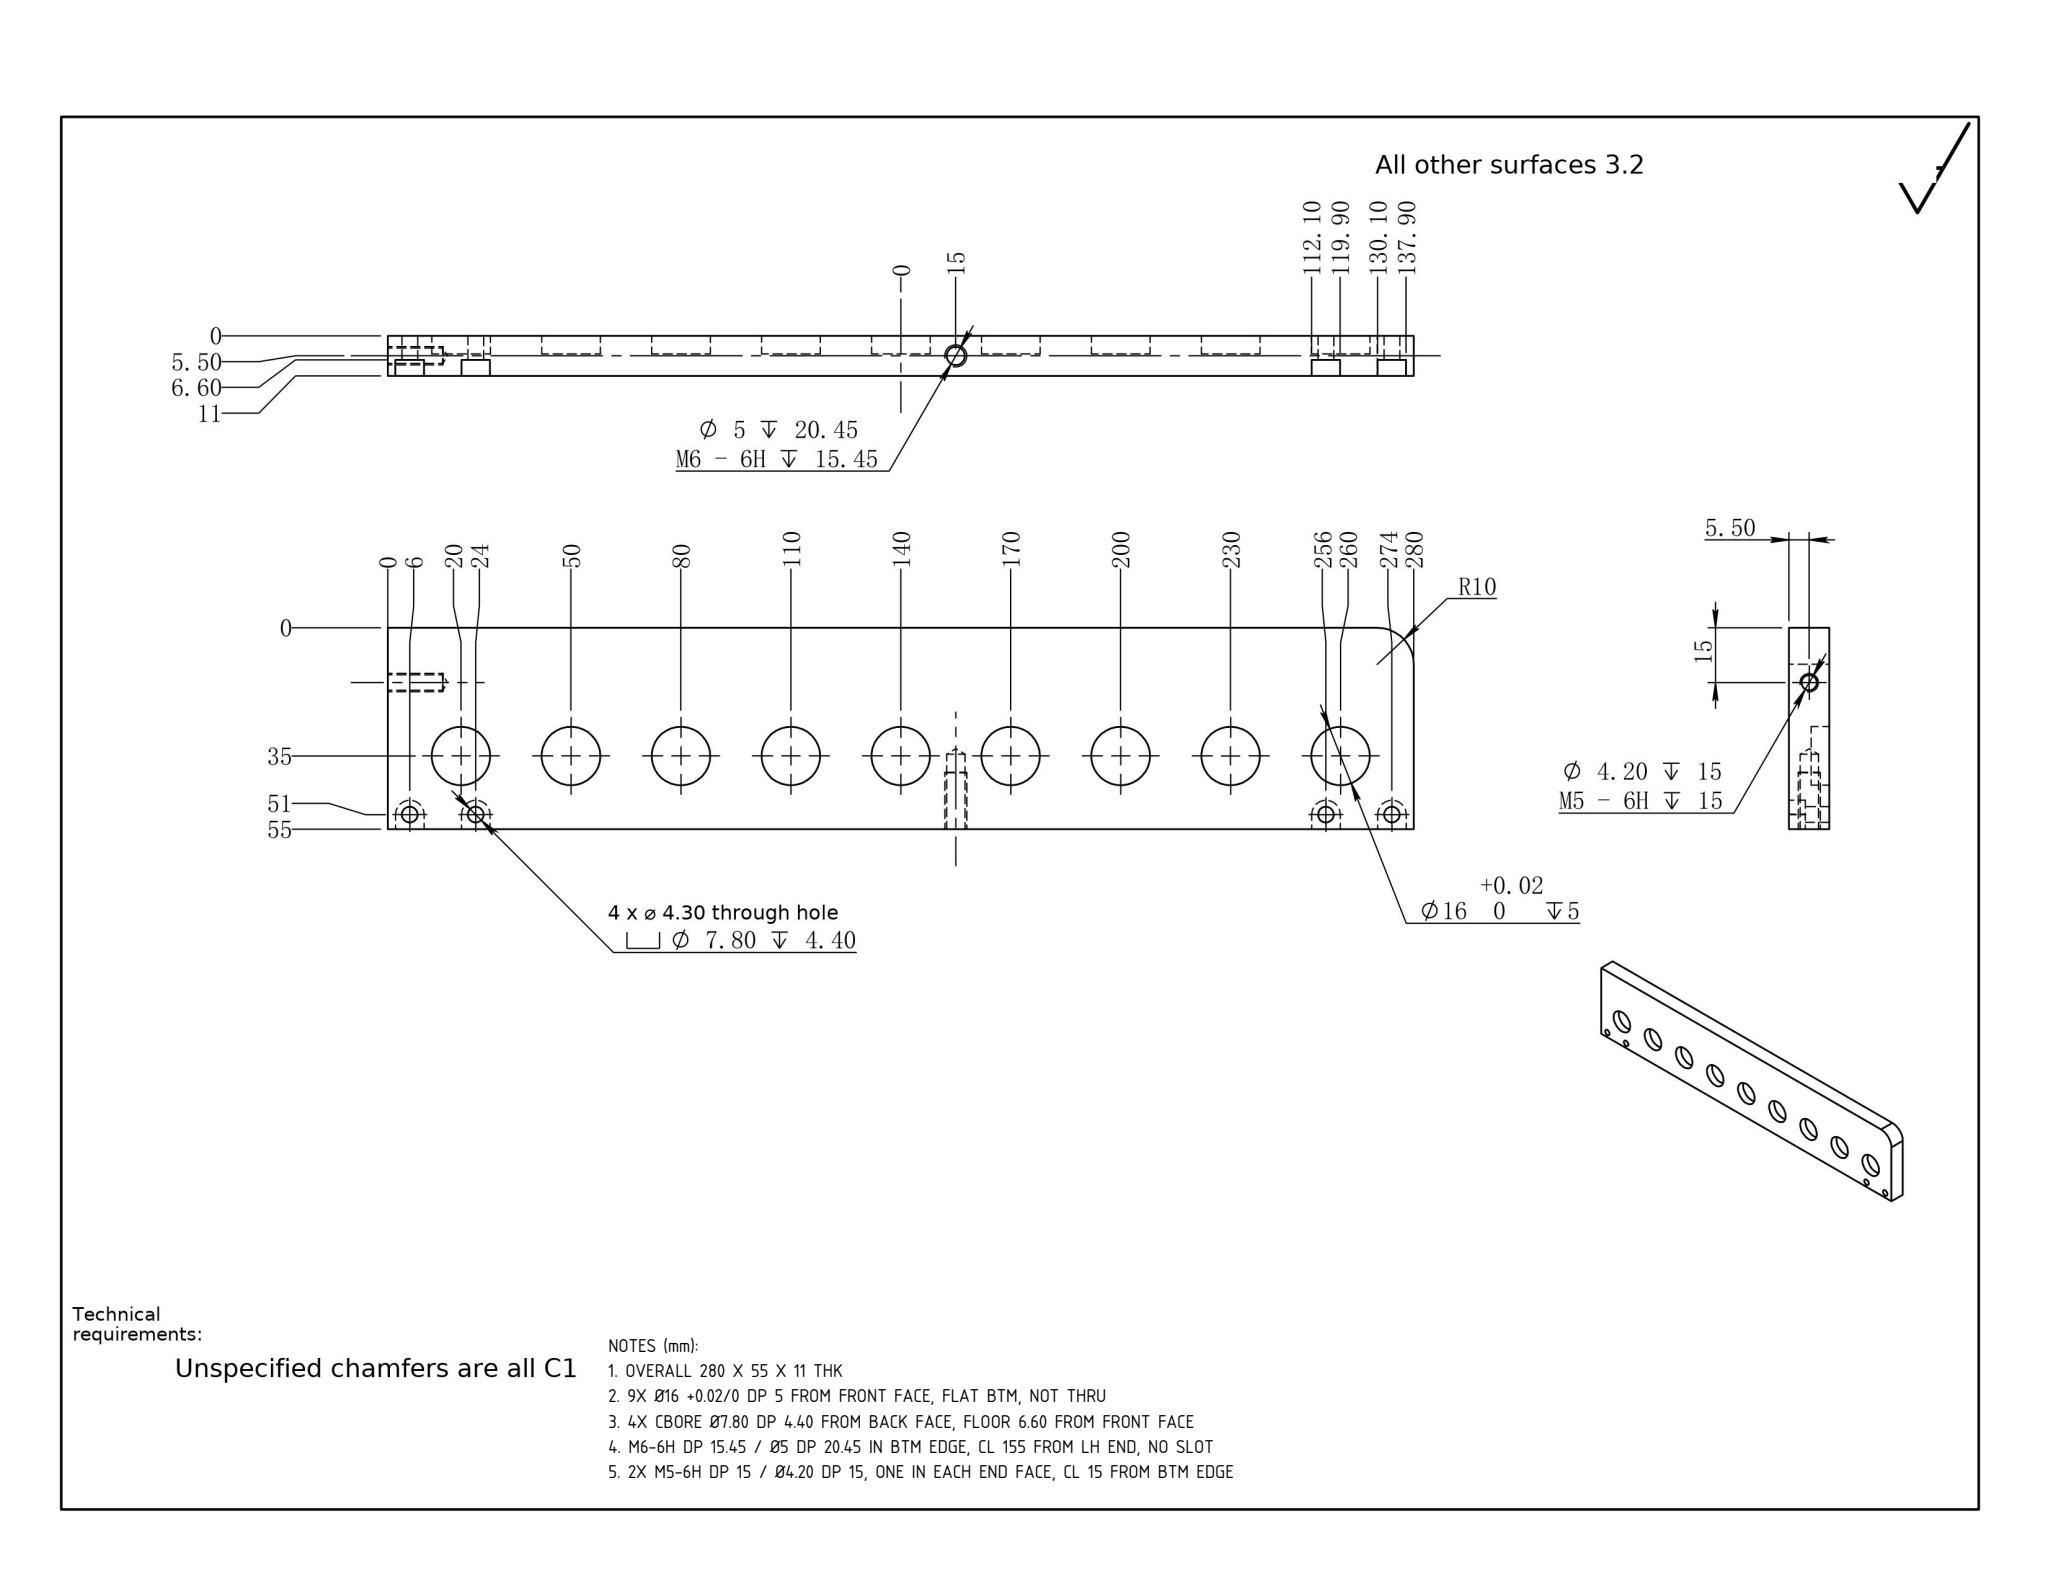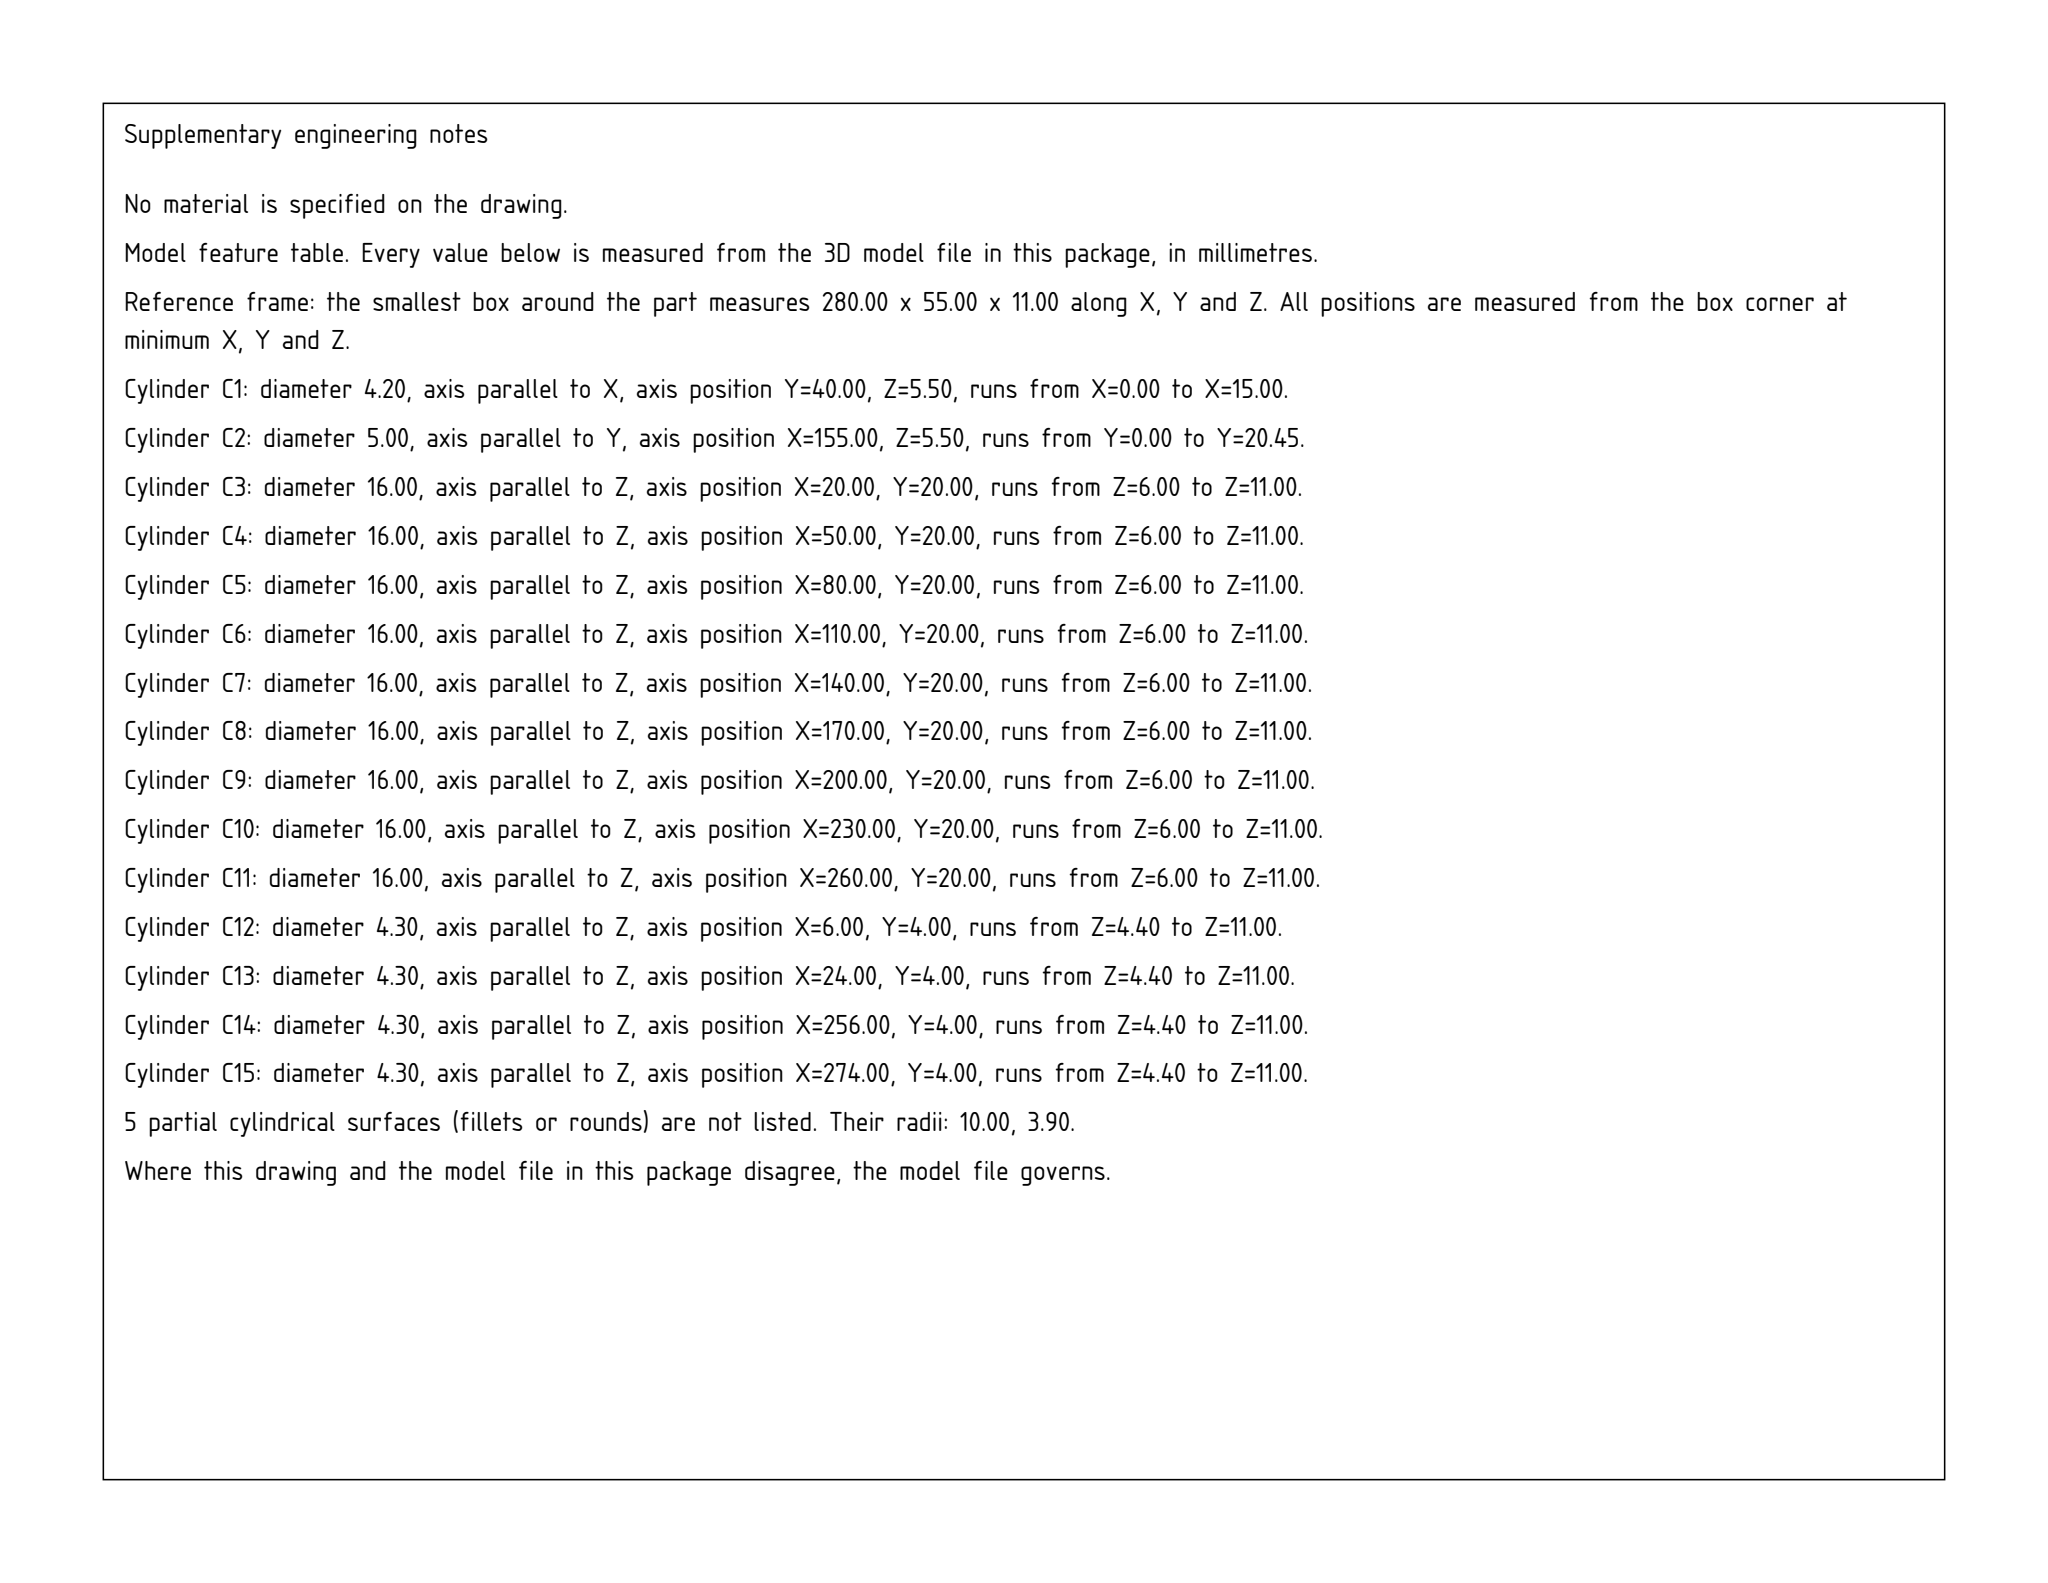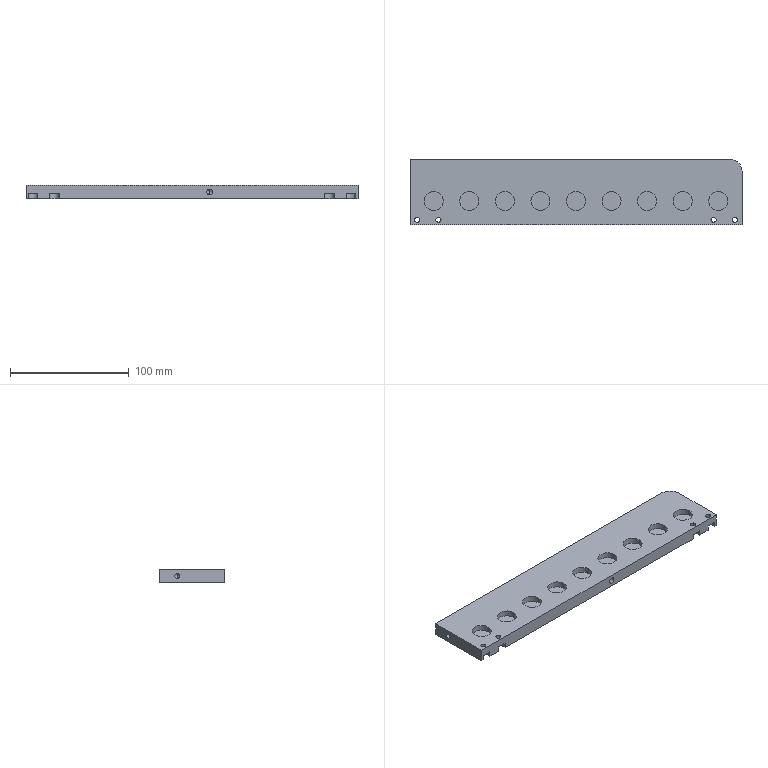Part | SolidWorks | mm | 1 solid | 66 faces | box 280 x 55 x 11 mm | volume 158138 mm3 | cylinder 35 | plane 27 | cone 4 | commonest cylinder face diameters 16 x18 4.3 x8 7.8 x4 4.2 x2 5 x2 20 x1
Drawing notes:
OVERALL 280 X 55 X 11 THK | from the solid: bbox_xyz [280.0, 55.0, 11.0]
9X Ø16 +0.02/0 DP 5 FROM FRONT FACE, FLAT BTM, NOT THRU | from the solid: Ø16 cyls at x=20,50,80,110,140,170,200,230,260 (y=20), len 5.0; 9 planar floors z=6.0; no smaller coaxial cyl
4X CBORE Ø7.80 DP 4.40 FROM BACK FACE, FLOOR 6.60 FROM FRONT FACE | from the solid: Ø7.8 z-cyls len 4.4 at x=6,24,256,274 (y=4); floor planes z=4.4 (4X) = 11-6.6; Ø4.3 thru cyls len 6.6
M6-6H DP 15.45 / Ø5 DP 20.45 IN BTM EDGE, CL 155 FROM LH END, NO SLOT | from the solid: single Ø5 y-axis cyl at x=155, z=5.5, len 20.45, 118° drill point; no pocket/slot geometry near x=140
2X M5-6H DP 15 / Ø4.20 DP 15, ONE IN EACH END FACE, CL 15 FROM BTM EDGE | from the solid: Ø4.2 x-axis cyls [null,40.0,5.5] len 15.0 count 2; 118° cones ref dia 4.2 x2; end faces x=0 and x=280; 55-40=15